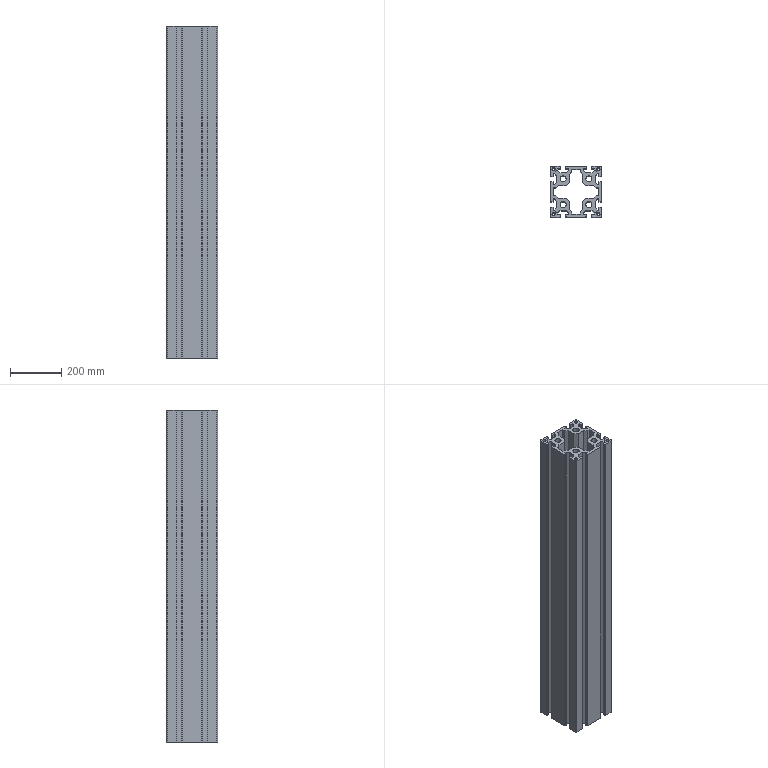Component | SolidWorks | AluminumProfile2-2 | 1 solid | 186 faces | box 200 x 200 x 1300 mm | volume 21413476 mm3 | plane 162 | cylinder 24 | commonest cylinder face diameters 12 x12 24 x8 10 x4
build123d program:
from build123d import *

# Parameters (mm, degrees)
SKETCH1_R           = 6
BOSS_EXTRUDE1_DEPTH = 650
SCALE1_SCALE        = 2


with BuildPart() as part:
    # Sketch1 → Boss-Extrude1 (new body)
    with BuildSketch(Plane(origin=(-310, 0, 0), x_dir=(0, -1, 0), z_dir=(-1, 0, 0))):
        with BuildLine():
            Line((45, 19.9), (45, 14))
            Line((45, 14), (41.657, 14))
            Line((41.657, 14), (37.2, 18.457))
            Line((37.2, 18.457), (37.2, 31.543))
            Line((37.2, 31.543), (41.657, 36))
            Line((41.657, 36), (45, 36))
            Line((45, 36), (45, 30.1))
            Line((45, 30.1), (49, 30.1))
            Line((49, 30.1), (49, 31.1))
            Line((49, 31.1), (50, 31.1))
            Line((50, 31.1), (50, 47.5))
            ThreePointArc((50, 47.5), (49.268, 49.268), (47.5, 50))
            Line((47.5, 50), (31.1, 50))
            Line((31.1, 50), (31.1, 49))
            Line((31.1, 49), (30.1, 49))
            Line((30.1, 49), (30.1, 45))
            Line((30.1, 45), (36, 45))
            Line((36, 45), (36, 41.657))
            Line((36, 41.657), (31.543, 37.2))
            Line((31.543, 37.2), (18.457, 37.2))
            Line((18.457, 37.2), (14, 41.657))
            Line((14, 41.657), (14, 45))
            Line((14, 45), (19.9, 45))
            Line((19.9, 45), (19.9, 49))
            Line((19.9, 49), (18.9, 49))
            Line((18.9, 49), (18.9, 50))
            Line((18.9, 50), (-18.9, 50))
            Line((-18.9, 50), (-18.9, 49))
            Line((-18.9, 49), (-19.9, 49))
            Line((-19.9, 49), (-19.9, 45))
            Line((-19.9, 45), (-14, 45))
            Line((-14, 45), (-14, 41.657))
            Line((-14, 41.657), (-18.457, 37.2))
            Line((-18.457, 37.2), (-31.543, 37.2))
            Line((-31.543, 37.2), (-36, 41.657))
            Line((-36, 41.657), (-36, 45))
            Line((-36, 45), (-30.1, 45))
            Line((-30.1, 45), (-30.1, 49))
            Line((-30.1, 49), (-31.1, 49))
            Line((-31.1, 49), (-31.1, 50))
            Line((-31.1, 50), (-47.5, 50))
            ThreePointArc((-47.5, 50), (-49.268, 49.268), (-50, 47.5))
            Line((-50, 47.5), (-50, 31.1))
            Line((-50, 31.1), (-49, 31.1))
            Line((-49, 31.1), (-49, 30.1))
            Line((-49, 30.1), (-45, 30.1))
            Line((-45, 30.1), (-45, 36))
            Line((-45, 36), (-41.657, 36))
            Line((-41.657, 36), (-37.2, 31.543))
            Line((-37.2, 31.543), (-37.2, 18.457))
            Line((-37.2, 18.457), (-41.657, 14))
            Line((-41.657, 14), (-45, 14))
            Line((-45, 14), (-45, 19.9))
            Line((-45, 19.9), (-49, 19.9))
            Line((-49, 19.9), (-49, 18.9))
            Line((-49, 18.9), (-50, 18.9))
            Line((-50, 18.9), (-50, -18.9))
            Line((-50, -18.9), (-49, -18.9))
            Line((-49, -18.9), (-49, -19.9))
            Line((-49, -19.9), (-45, -19.9))
            Line((-45, -19.9), (-45, -14))
            Line((-45, -14), (-41.657, -14))
            Line((-41.657, -14), (-37.2, -18.457))
            Line((-37.2, -18.457), (-37.2, -31.543))
            Line((-37.2, -31.543), (-41.657, -36))
            Line((-41.657, -36), (-45, -36))
            Line((-45, -36), (-45, -30.1))
            Line((-45, -30.1), (-49, -30.1))
            Line((-49, -30.1), (-49, -31.1))
            Line((-49, -31.1), (-50, -31.1))
            Line((-50, -31.1), (-50, -47.5))
            ThreePointArc((-50, -47.5), (-49.268, -49.268), (-47.5, -50))
            Line((-47.5, -50), (-31.1, -50))
            Line((-31.1, -50), (-31.1, -49))
            Line((-31.1, -49), (-30.1, -49))
            Line((-30.1, -49), (-30.1, -45))
            Line((-30.1, -45), (-36, -45))
            Line((-36, -45), (-36, -41.657))
            Line((-36, -41.657), (-31.543, -37.2))
            Line((-31.543, -37.2), (-18.457, -37.2))
            Line((-18.457, -37.2), (-14, -41.657))
            Line((-14, -41.657), (-14, -45))
            Line((-14, -45), (-19.9, -45))
            Line((-19.9, -45), (-19.9, -49))
            Line((-19.9, -49), (-18.9, -49))
            Line((-18.9, -49), (-18.9, -50))
            Line((-18.9, -50), (18.9, -50))
            Line((18.9, -50), (18.9, -49))
            Line((18.9, -49), (19.9, -49))
            Line((19.9, -49), (19.9, -45))
            Line((19.9, -45), (14, -45))
            Line((14, -45), (14, -41.657))
            Line((14, -41.657), (18.457, -37.2))
            Line((18.457, -37.2), (31.543, -37.2))
            Line((31.543, -37.2), (36, -41.657))
            Line((36, -41.657), (36, -45))
            Line((36, -45), (30.1, -45))
            Line((30.1, -45), (30.1, -49))
            Line((30.1, -49), (31.1, -49))
            Line((31.1, -49), (31.1, -50))
            Line((31.1, -50), (47.5, -50))
            ThreePointArc((47.5, -50), (49.268, -49.268), (50, -47.5))
            Line((50, -47.5), (50, -31.1))
            Line((50, -31.1), (49, -31.1))
            Line((49, -31.1), (49, -30.1))
            Line((49, -30.1), (45, -30.1))
            Line((45, -30.1), (45, -36))
            Line((45, -36), (41.657, -36))
            Line((41.657, -36), (37.2, -31.543))
            Line((37.2, -31.543), (37.2, -18.457))
            Line((37.2, -18.457), (41.657, -14))
            Line((41.657, -14), (45, -14))
            Line((45, -14), (45, -19.9))
            Line((45, -19.9), (49, -19.9))
            Line((49, -19.9), (49, -18.9))
            Line((49, -18.9), (50, -18.9))
            Line((50, -18.9), (50, 18.9))
            Line((50, 18.9), (49, 18.9))
            Line((49, 18.9), (49, 19.9))
            Line((49, 19.9), (45, 19.9))
        make_face()
        with Locations(Location((25, 25, 0), (0, 0, 180))):
            Circle(SKETCH1_R, mode=Mode.SUBTRACT)
        with Locations(Location((25, -25, 0), (0, 0, 180))):
            Circle(SKETCH1_R, mode=Mode.SUBTRACT)
        with Locations(Location((-25, 25, 0), (0, 0, 180))):
            Circle(SKETCH1_R, mode=Mode.SUBTRACT)
        with Locations(Location((-25, -25, 0), (0, 0, 180))):
            Circle(SKETCH1_R, mode=Mode.SUBTRACT)
        with BuildLine():
            Line((38.981, -40.678), (40.678, -38.981))
            Line((40.678, -38.981), (42.904, -41.207))
            ThreePointArc((42.904, -41.207), (46.121, -46.121), (41.207, -42.904))
            Line((41.207, -42.904), (38.981, -40.678))
        make_face(mode=Mode.SUBTRACT)
        with BuildLine():
            Line((-40.678, -38.981), (-38.981, -40.678))
            Line((-38.981, -40.678), (-41.207, -42.904))
            ThreePointArc((-41.207, -42.904), (-46.121, -46.121), (-42.904, -41.207))
            Line((-42.904, -41.207), (-40.678, -38.981))
        make_face(mode=Mode.SUBTRACT)
        Polygon((34.372, 12.8), (39.172, 8), (44, 8), (44, -8), (39.172, -8), (34.372, -12.8), (18.8, -12.8), (12.8, -18.8), (12.8, -34.372), (8, -39.172), (8, -44), (-8, -44), (-8, -39.172), (-12.8, -34.372), (-12.8, -18.8), (-18.8, -12.8), (-34.372, -12.8), (-39.172, -8), (-44, -8), (-44, 8), (-39.172, 8), (-34.372, 12.8), (-18.8, 12.8), (-12.8, 18.8), (-12.8, 34.372), (-8, 39.172), (-8, 44), (8, 44), (8, 39.172), (12.8, 34.372), (12.8, 18.8), (18.8, 12.8), align=None, mode=Mode.SUBTRACT)
        with BuildLine():
            Line((42.904, 41.207), (40.678, 38.981))
            Line((40.678, 38.981), (38.981, 40.678))
            Line((38.981, 40.678), (41.207, 42.904))
            ThreePointArc((41.207, 42.904), (46.121, 46.121), (42.904, 41.207))
        make_face(mode=Mode.SUBTRACT)
        with BuildLine():
            Line((-41.207, 42.904), (-38.981, 40.678))
            Line((-38.981, 40.678), (-40.678, 38.981))
            Line((-40.678, 38.981), (-42.904, 41.207))
            ThreePointArc((-42.904, 41.207), (-46.121, 46.121), (-41.207, 42.904))
        make_face(mode=Mode.SUBTRACT)
    extrude(amount=-BOSS_EXTRUDE1_DEPTH)


with BuildPart() as part_1:
    # Scale1: scaled about (15, 0, -0)
    add(part.part.scale(SCALE1_SCALE).moved(Location((-15, 0, 0))))


solid = part_1.part

# Placed as in the assembly
solid = solid.moved(Location((1286, -931, 510), (0, 90, 0)))